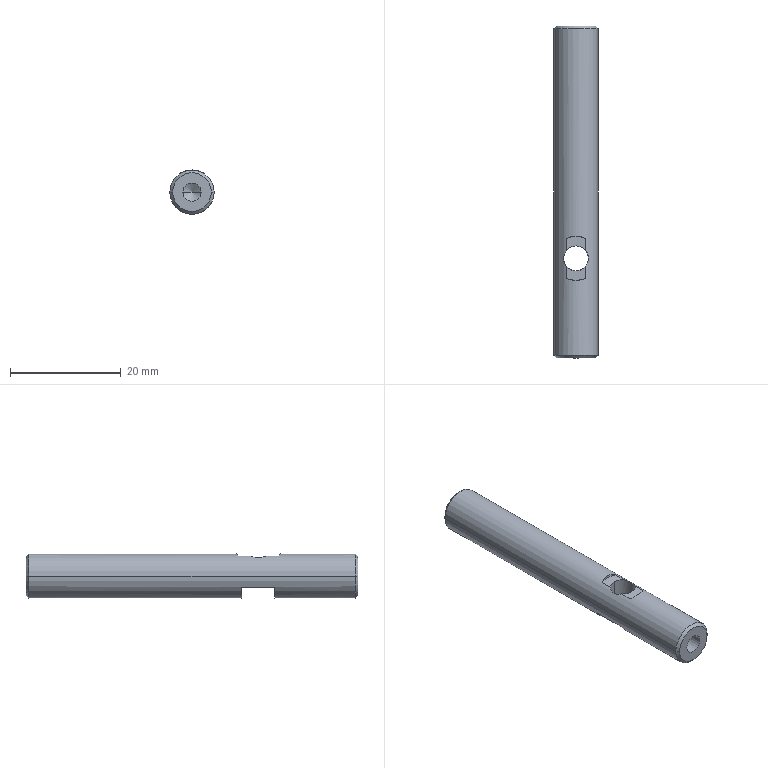Component | SolidWorks | 002MaterialPickingModuleA-1_004SidePlugModule-1_J-017-1 | 1 solid | 26 faces | box 8 x 60 x 8 mm | volume 2727 mm3 | cylinder 11 | cone 8 | plane 7 | commonest cylinder face diameters 8 x5 3.3 x2 4.5 x2 2.5 x2 | material 45
build123d program:
from build123d import *

# Parameters (mm, degrees)
SKETCH1_R             = 4
BOSS_EXTRUDE1_DEPTH   = 48
M3_TAPPED_HOLE1_D     = 2.5
M3_TAPPED_HOLE1_DEPTH = 7.5
M3_TAPPED_HOLE1_TIP   = 0.7511
CHAMFER1_SIZE         = 0.5
SKETCH6_W             = 15
SKETCH6_H             = 6
CUT_EXTRUDE1_DEPTH    = 2
SKETCH9_R             = 4
BOSS_EXTRUDE2_DEPTH   = 12
CHAMFER2_SIZE         = 0.5
M4_TAPPED_HOLE1_D     = 3.3
M4_TAPPED_HOLE1_DEPTH = 10.1
M4_TAPPED_HOLE1_TIP   = 0.9914


with BuildPart() as part:
    # Sketch1 → Boss-Extrude1 (new body)
    with BuildSketch(Plane.XY):
        Circle(SKETCH1_R)
    extrude(amount=BOSS_EXTRUDE1_DEPTH)

    # M3 Tapped Hole1
    with Locations(Plane(origin=(0, 0, 0), x_dir=(-1, 0, 0), z_dir=(0, 0, -1))):
        with Locations((0, 0)):
            Hole(M3_TAPPED_HOLE1_D / 2, depth=M3_TAPPED_HOLE1_DEPTH)
            with Locations((0, 0, -(M3_TAPPED_HOLE1_DEPTH + M3_TAPPED_HOLE1_TIP / 2))):  # 118° drill point
                Cone(0, M3_TAPPED_HOLE1_D / 2, M3_TAPPED_HOLE1_TIP, mode=Mode.SUBTRACT)

    # Chamfer1
    chamfer1_edges = [part.edges().sort_by_distance(p)[0] for p in [
        (-4, 0, 0),
    ]]
    chamfer(chamfer1_edges, length=CHAMFER1_SIZE)

    # Sketch6 → Cut-Extrude1 (cut)
    with BuildSketch(Plane(origin=(0, 4, 0), x_dir=(1, 0, 0), z_dir=(0, 1, 0))):
        with Locations((0, -42)):
            Rectangle(SKETCH6_W, SKETCH6_H)
    extrude(amount=-CUT_EXTRUDE1_DEPTH, mode=Mode.SUBTRACT)

    # Sketch8 → M4 Hex Socket Head Cap Screw CBORE1 (revolve, cut)
    with BuildSketch(Plane(origin=(0, -8, 42), x_dir=(0, 0, -1), z_dir=(1, 0, 0))):
        Polygon((0, 0), (0, 12), (2.25, 12), (2.25, 4.4), (4, 4.4), (4, 0.025), (4.025, 0), align=None)
    revolve(axis=Axis((0, -14.35, 42), (0, 1, 0)), mode=Mode.SUBTRACT)

    # Sketch9 → Boss-Extrude2 (add)
    with BuildSketch(Plane.XY.offset(48)):
        Circle(SKETCH9_R)
    extrude(amount=BOSS_EXTRUDE2_DEPTH)

    # Chamfer2
    chamfer2_edges = [part.edges().sort_by_distance(p)[0] for p in [
        (-4, 0, 60),
    ]]
    chamfer(chamfer2_edges, length=CHAMFER2_SIZE)

    # M4 Tapped Hole1
    with Locations(Plane.XY.offset(60)):
        with Locations((0, 0)):
            Hole(M4_TAPPED_HOLE1_D / 2, depth=M4_TAPPED_HOLE1_DEPTH)
            with Locations((0, 0, -(M4_TAPPED_HOLE1_DEPTH + M4_TAPPED_HOLE1_TIP / 2))):  # 118° drill point
                Cone(0, M4_TAPPED_HOLE1_D / 2, M4_TAPPED_HOLE1_TIP, mode=Mode.SUBTRACT)


solid = part.part

# Placed as in the assembly
solid = solid.moved(Location((195.325, 338.019, 464.731), (90, 0, -180)))
STEP:
#1=CARTESIAN_POINT('',(7.755,11.343,18.296));
#2=VERTEX_POINT('',#1);
#3=CARTESIAN_POINT('',(7.625,11.343,18.296));
#4=VERTEX_POINT('',#3);
#5=CARTESIAN_POINT('',(7.69,11.343,18.296));
#6=DIRECTION('',(0.,-1.,-0.));
#7=DIRECTION('',(-1.,0.,0.));
#8=AXIS2_PLACEMENT_3D('',#5,#6,#7);
#9=CIRCLE('',#8,0.06496);
#10=EDGE_CURVE('',#2,#4,#9,.T.);
#11=ORIENTED_EDGE('',*,*,#10,.F.);
#12=CARTESIAN_POINT('',(7.755,10.946,18.296));
#13=VERTEX_POINT('',#12);
#14=CARTESIAN_POINT('',(7.755,10.946,18.296));
#15=DIRECTION('',(0.,-1.,-0.));
#16=VECTOR('',#15,39.37);
#17=LINE('',#14,#16);
#18=EDGE_CURVE('',#2,#13,#17,.T.);
#19=ORIENTED_EDGE('',*,*,#18,.T.);
#20=CARTESIAN_POINT('',(7.625,10.946,18.296));
#21=VERTEX_POINT('',#20);
#22=CARTESIAN_POINT('',(7.69,10.946,18.296));
#23=DIRECTION('',(0.,-1.,-0.));
#24=DIRECTION('',(-1.,0.,0.));
#25=AXIS2_PLACEMENT_3D('',#22,#23,#24);
#26=CIRCLE('',#25,0.06496);
#27=EDGE_CURVE('',#13,#21,#26,.T.);
#28=ORIENTED_EDGE('',*,*,#27,.T.);
#29=CARTESIAN_POINT('',(7.625,10.946,18.296));
#30=DIRECTION('',(0.,-1.,-0.));
#31=VECTOR('',#30,39.37);
#32=LINE('',#29,#31);
#33=EDGE_CURVE('',#4,#21,#32,.T.);
#34=ORIENTED_EDGE('',*,*,#33,.F.);
#35=EDGE_LOOP('',(#11,#19,#28,#34));
#36=FACE_OUTER_BOUND('',#35,.T.);
#37=CARTESIAN_POINT('',(7.69,10.946,18.296));
#38=DIRECTION('',(0.,-1.,-0.));
#39=DIRECTION('',(-1.,0.,0.));
#40=AXIS2_PLACEMENT_3D('',#37,#38,#39);
#41=CYLINDRICAL_SURFACE('',#40,0.06496);
#42=ADVANCED_FACE('',(#36),#41,.F.);
#43=CARTESIAN_POINT('',(7.69,11.382,18.296));
#44=VERTEX_POINT('',#43);
#45=CARTESIAN_POINT('',(7.625,11.343,18.296));
#46=DIRECTION('',(-0.8572,-0.515,0.));
#47=VECTOR('',#46,39.37);
#48=LINE('',#45,#47);
#49=EDGE_CURVE('',#44,#4,#48,.T.);
#50=ORIENTED_EDGE('',*,*,#49,.F.);
#51=CARTESIAN_POINT('',(7.755,11.343,18.296));
#52=DIRECTION('',(0.8572,-0.515,-0.));
#53=VECTOR('',#52,39.37);
#54=LINE('',#51,#53);
#55=EDGE_CURVE('',#44,#2,#54,.T.);
#56=ORIENTED_EDGE('',*,*,#55,.T.);
#57=ORIENTED_EDGE('',*,*,#10,.T.);
#58=EDGE_LOOP('',(#50,#56,#57));
#59=FACE_OUTER_BOUND('',#58,.T.);
#60=CARTESIAN_POINT('',(7.69,11.343,18.296));
#61=DIRECTION('',(0.,-1.,-0.));
#62=DIRECTION('',(-1.,0.,0.));
#63=AXIS2_PLACEMENT_3D('',#60,#61,#62);
#64=CONICAL_SURFACE('',#63,0.06496,1.03);
#65=ADVANCED_FACE('',(#59),#64,.F.);
#66=CARTESIAN_POINT('',(7.552,10.946,18.296));
#67=VERTEX_POINT('',#66);
#68=CARTESIAN_POINT('',(7.828,10.946,18.296));
#69=VERTEX_POINT('',#68);
#70=CARTESIAN_POINT('',(7.69,10.946,18.296));
#71=DIRECTION('',(0.,-1.,-0.));
#72=DIRECTION('',(-1.,0.,0.));
#73=AXIS2_PLACEMENT_3D('',#70,#71,#72);
#74=CIRCLE('',#73,0.1378);
#75=EDGE_CURVE('',#67,#69,#74,.T.);
#76=ORIENTED_EDGE('',*,*,#75,.F.);
#77=CARTESIAN_POINT('',(7.532,10.965,18.296));
#78=VERTEX_POINT('',#77);
#79=CARTESIAN_POINT('',(7.552,10.946,18.296));
#80=DIRECTION('',(-0.7071,0.7071,0.));
#81=VECTOR('',#80,39.37);
#82=LINE('',#79,#81);
#83=EDGE_CURVE('',#67,#78,#82,.T.);
#84=ORIENTED_EDGE('',*,*,#83,.T.);
#85=CARTESIAN_POINT('',(7.847,10.965,18.296));
#86=VERTEX_POINT('',#85);
#87=CARTESIAN_POINT('',(7.69,10.965,18.296));
#88=DIRECTION('',(-0.,1.,0.));
#89=DIRECTION('',(-1.,0.,0.));
#90=AXIS2_PLACEMENT_3D('',#87,#88,#89);
#91=CIRCLE('',#90,0.1575);
#92=EDGE_CURVE('',#86,#78,#91,.T.);
#93=ORIENTED_EDGE('',*,*,#92,.F.);
#94=CARTESIAN_POINT('',(7.828,10.946,18.296));
#95=DIRECTION('',(0.7071,0.7071,-0.));
#96=VECTOR('',#95,39.37);
#97=LINE('',#94,#96);
#98=EDGE_CURVE('',#69,#86,#97,.T.);
#99=ORIENTED_EDGE('',*,*,#98,.F.);
#100=EDGE_LOOP('',(#76,#84,#93,#99));
#101=FACE_OUTER_BOUND('',#100,.T.);
#102=CARTESIAN_POINT('',(7.69,10.946,18.296));
#103=DIRECTION('',(-0.,1.,0.));
#104=DIRECTION('',(1.,0.,0.));
#105=AXIS2_PLACEMENT_3D('',#102,#103,#104);
#106=CONICAL_SURFACE('',#105,0.1378,0.7854);
#107=ADVANCED_FACE('',(#101),#106,.T.);
#108=CARTESIAN_POINT('',(7.69,11.743,18.218));
#109=VERTEX_POINT('',#108);
#110=CARTESIAN_POINT('',(7.69,11.566,18.218));
#111=VERTEX_POINT('',#110);
#112=CARTESIAN_POINT('',(7.69,11.654,18.218));
#113=DIRECTION('',(-0.,0.,-1.));
#114=DIRECTION('',(0.,-1.,0.));
#115=AXIS2_PLACEMENT_3D('',#112,#113,#114);
#116=CIRCLE('',#115,0.08858);
#117=EDGE_CURVE('',#109,#111,#116,.T.);
#118=ORIENTED_EDGE('',*,*,#117,.T.);
#119=CARTESIAN_POINT('',(7.69,11.566,18.438));
#120=VERTEX_POINT('',#119);
#121=CARTESIAN_POINT('',(7.69,11.566,18.611));
#122=DIRECTION('',(0.,-0.,1.));
#123=VECTOR('',#122,39.37);
#124=LINE('',#121,#123);
#125=EDGE_CURVE('',#111,#120,#124,.T.);
#126=ORIENTED_EDGE('',*,*,#125,.T.);
#127=CARTESIAN_POINT('',(7.759,11.598,18.438));
#128=VERTEX_POINT('',#127);
#129=CARTESIAN_POINT('',(7.69,11.654,18.438));
#130=DIRECTION('',(0.,-0.,1.));
#131=DIRECTION('',(0.,1.,0.));
#132=AXIS2_PLACEMENT_3D('',#129,#130,#131);
#133=CIRCLE('',#132,0.08858);
#134=EDGE_CURVE('',#120,#128,#133,.T.);
#135=ORIENTED_EDGE('',*,*,#134,.T.);
#136=CARTESIAN_POINT('',(7.759,11.71,18.438));
#137=VERTEX_POINT('',#136);
#138=CARTESIAN_POINT('',(7.759,11.71,18.438));
#139=CARTESIAN_POINT('',(7.765,11.703,18.435));
#140=CARTESIAN_POINT('',(7.77,11.694,18.432));
#141=CARTESIAN_POINT('',(7.775,11.68,18.429));
#142=CARTESIAN_POINT('',(7.776,11.675,18.428));
#143=CARTESIAN_POINT('',(7.778,11.665,18.427));
#144=CARTESIAN_POINT('',(7.779,11.66,18.427));
#145=CARTESIAN_POINT('',(7.779,11.649,18.427));
#146=CARTESIAN_POINT('',(7.778,11.644,18.427));
#147=CARTESIAN_POINT('',(7.776,11.634,18.428));
#148=CARTESIAN_POINT('',(7.775,11.629,18.429));
#149=CARTESIAN_POINT('',(7.77,11.615,18.432));
#150=CARTESIAN_POINT('',(7.765,11.606,18.435));
#151=CARTESIAN_POINT('',(7.759,11.598,18.438));
#152=B_SPLINE_CURVE_WITH_KNOTS('',3,(#138,#139,#140,#141,#142,#143,#144,#145,#146,#147,#148,#149,#150,#151),.UNSPECIFIED.,.F.,.F.,(4,2,2,2,2,2,4),(0.,0.0007826,0.001174,0.001565,0.001957,0.002348,0.00313),.UNSPECIFIED.);
#153=EDGE_CURVE('',#137,#128,#152,.T.);
#154=ORIENTED_EDGE('',*,*,#153,.F.);
#155=CARTESIAN_POINT('',(7.69,11.743,18.438));
#156=VERTEX_POINT('',#155);
#157=CARTESIAN_POINT('',(7.69,11.654,18.438));
#158=DIRECTION('',(0.,-0.,1.));
#159=DIRECTION('',(0.,1.,0.));
#160=AXIS2_PLACEMENT_3D('',#157,#158,#159);
#161=CIRCLE('',#160,0.08858);
#162=EDGE_CURVE('',#137,#156,#161,.T.);
#163=ORIENTED_EDGE('',*,*,#162,.T.);
#164=CARTESIAN_POINT('',(7.69,11.743,18.611));
#165=DIRECTION('',(0.,-0.,1.));
#166=VECTOR('',#165,39.37);
#167=LINE('',#164,#166);
#168=EDGE_CURVE('',#109,#156,#167,.T.);
#169=ORIENTED_EDGE('',*,*,#168,.F.);
#170=EDGE_LOOP('',(#118,#126,#135,#154,#163,#169));
#171=FACE_OUTER_BOUND('',#170,.T.);
#172=CARTESIAN_POINT('',(7.69,11.654,18.611));
#173=DIRECTION('',(0.,-0.,1.));
#174=DIRECTION('',(0.,1.,0.));
#175=AXIS2_PLACEMENT_3D('',#172,#173,#174);
#176=CYLINDRICAL_SURFACE('',#175,0.08858);
#177=ADVANCED_FACE('',(#171),#176,.F.);
#178=CARTESIAN_POINT('',(7.69,11.812,18.438));
#179=VERTEX_POINT('',#178);
#180=CARTESIAN_POINT('',(7.621,11.796,18.438));
#181=VERTEX_POINT('',#180);
#182=CARTESIAN_POINT('',(7.69,11.654,18.438));
#183=DIRECTION('',(0.,-0.,1.));
#184=DIRECTION('',(0.,1.,0.));
#185=AXIS2_PLACEMENT_3D('',#182,#183,#184);
#186=CIRCLE('',#185,0.1575);
#187=EDGE_CURVE('',#179,#181,#186,.T.);
#188=ORIENTED_EDGE('',*,*,#187,.F.);
#189=CARTESIAN_POINT('',(7.69,11.812,18.454));
#190=VERTEX_POINT('',#189);
#191=CARTESIAN_POINT('',(7.69,11.812,18.611));
#192=DIRECTION('',(0.,-0.,1.));
#193=VECTOR('',#192,39.37);
#194=LINE('',#191,#193);
#195=EDGE_CURVE('',#179,#190,#194,.T.);
#196=ORIENTED_EDGE('',*,*,#195,.T.);
#197=CARTESIAN_POINT('',(7.621,11.796,18.438));
#198=CARTESIAN_POINT('',(7.643,11.806,18.449));
#199=CARTESIAN_POINT('',(7.666,11.812,18.454));
#200=CARTESIAN_POINT('',(7.69,11.812,18.454));
#201=(BOUNDED_CURVE()B_SPLINE_CURVE(3,(#197,#198,#199,#200),.UNSPECIFIED.,.F.,.T.)B_SPLINE_CURVE_WITH_KNOTS((4,4),(5.832,6.283),.UNSPECIFIED.)CURVE()GEOMETRIC_REPRESENTATION_ITEM()RATIONAL_B_SPLINE_CURVE((1.,0.9831,0.9831,1.))REPRESENTATION_ITEM(''));
#202=EDGE_CURVE('',#181,#190,#201,.T.);
#203=ORIENTED_EDGE('',*,*,#202,.F.);
#204=EDGE_LOOP('',(#188,#196,#203));
#205=FACE_OUTER_BOUND('',#204,.T.);
#206=CARTESIAN_POINT('',(7.69,11.654,18.611));
#207=DIRECTION('',(0.,-0.,1.));
#208=DIRECTION('',(0.,1.,0.));
#209=AXIS2_PLACEMENT_3D('',#206,#207,#208);
#210=CYLINDRICAL_SURFACE('',#209,0.1575);
#211=ADVANCED_FACE('',(#205),#210,.F.);
#212=CARTESIAN_POINT('',(7.828,13.308,18.296));
#213=VERTEX_POINT('',#212);
#214=CARTESIAN_POINT('',(7.552,13.308,18.296));
#215=VERTEX_POINT('',#214);
#216=CARTESIAN_POINT('',(7.69,13.308,18.296));
#217=DIRECTION('',(-0.,1.,0.));
#218=DIRECTION('',(-1.,0.,0.));
#219=AXIS2_PLACEMENT_3D('',#216,#217,#218);
#220=CIRCLE('',#219,0.1378);
#221=EDGE_CURVE('',#213,#215,#220,.T.);
#222=ORIENTED_EDGE('',*,*,#221,.F.);
#223=CARTESIAN_POINT('',(7.847,13.288,18.296));
#224=VERTEX_POINT('',#223);
#225=CARTESIAN_POINT('',(7.847,13.288,18.296));
#226=DIRECTION('',(0.7071,-0.7071,-0.));
#227=VECTOR('',#226,39.37);
#228=LINE('',#225,#227);
#229=EDGE_CURVE('',#213,#224,#228,.T.);
#230=ORIENTED_EDGE('',*,*,#229,.T.);
#231=CARTESIAN_POINT('',(7.532,13.288,18.296));
#232=VERTEX_POINT('',#231);
#233=CARTESIAN_POINT('',(7.69,13.288,18.296));
#234=DIRECTION('',(0.,-1.,-0.));
#235=DIRECTION('',(-1.,0.,0.));
#236=AXIS2_PLACEMENT_3D('',#233,#234,#235);
#237=CIRCLE('',#236,0.1575);
#238=EDGE_CURVE('',#232,#224,#237,.T.);
#239=ORIENTED_EDGE('',*,*,#238,.F.);
#240=CARTESIAN_POINT('',(7.532,13.288,18.296));
#241=DIRECTION('',(-0.7071,-0.7071,0.));
#242=VECTOR('',#241,39.37);
#243=LINE('',#240,#242);
#244=EDGE_CURVE('',#215,#232,#243,.T.);
#245=ORIENTED_EDGE('',*,*,#244,.F.);
#246=EDGE_LOOP('',(#222,#230,#239,#245));
#247=FACE_OUTER_BOUND('',#246,.T.);
#248=CARTESIAN_POINT('',(7.69,13.288,18.296));
#249=DIRECTION('',(0.,-1.,-0.));
#250=DIRECTION('',(-1.,0.,0.));
#251=AXIS2_PLACEMENT_3D('',#248,#249,#250);
#252=CONICAL_SURFACE('',#251,0.1575,0.7854);
#253=ADVANCED_FACE('',(#247),#252,.T.);
#254=CARTESIAN_POINT('',(7.641,13.013,18.296));
#255=VERTEX_POINT('',#254);
#256=CARTESIAN_POINT('',(7.739,13.013,18.296));
#257=VERTEX_POINT('',#256);
#258=CARTESIAN_POINT('',(7.69,13.013,18.296));
#259=DIRECTION('',(-0.,1.,0.));
#260=DIRECTION('',(1.,0.,0.));
#261=AXIS2_PLACEMENT_3D('',#258,#259,#260);
#262=CIRCLE('',#261,0.04921);
#263=EDGE_CURVE('',#255,#257,#262,.T.);
#264=ORIENTED_EDGE('',*,*,#263,.F.);
#265=CARTESIAN_POINT('',(7.641,13.308,18.296));
#266=VERTEX_POINT('',#265);
#267=CARTESIAN_POINT('',(7.641,13.308,18.296));
#268=DIRECTION('',(-0.,1.,0.));
#269=VECTOR('',#268,39.37);
#270=LINE('',#267,#269);
#271=EDGE_CURVE('',#255,#266,#270,.T.);
#272=ORIENTED_EDGE('',*,*,#271,.T.);
#273=CARTESIAN_POINT('',(7.739,13.308,18.296));
#274=VERTEX_POINT('',#273);
#275=CARTESIAN_POINT('',(7.69,13.308,18.296));
#276=DIRECTION('',(-0.,1.,0.));
#277=DIRECTION('',(1.,0.,0.));
#278=AXIS2_PLACEMENT_3D('',#275,#276,#277);
#279=CIRCLE('',#278,0.04921);
#280=EDGE_CURVE('',#266,#274,#279,.T.);
#281=ORIENTED_EDGE('',*,*,#280,.T.);
#282=CARTESIAN_POINT('',(7.739,13.308,18.296));
#283=DIRECTION('',(-0.,1.,0.));
#284=VECTOR('',#283,39.37);
#285=LINE('',#282,#284);
#286=EDGE_CURVE('',#257,#274,#285,.T.);
#287=ORIENTED_EDGE('',*,*,#286,.F.);
#288=EDGE_LOOP('',(#264,#272,#281,#287));
#289=FACE_OUTER_BOUND('',#288,.T.);
#290=CARTESIAN_POINT('',(7.69,13.308,18.296));
#291=DIRECTION('',(-0.,1.,0.));
#292=DIRECTION('',(1.,0.,0.));
#293=AXIS2_PLACEMENT_3D('',#290,#291,#292);
#294=CYLINDRICAL_SURFACE('',#293,0.04921);
#295=ADVANCED_FACE('',(#289),#294,.F.);
#296=CARTESIAN_POINT('',(7.69,12.983,18.296));
#297=VERTEX_POINT('',#296);
#298=CARTESIAN_POINT('',(7.739,13.013,18.296));
#299=DIRECTION('',(0.8572,0.515,-0.));
#300=VECTOR('',#299,39.37);
#301=LINE('',#298,#300);
#302=EDGE_CURVE('',#297,#257,#301,.T.);
#303=ORIENTED_EDGE('',*,*,#302,.F.);
#304=CARTESIAN_POINT('',(7.641,13.013,18.296));
#305=DIRECTION('',(-0.8572,0.515,0.));
#306=VECTOR('',#305,39.37);
#307=LINE('',#304,#306);
#308=EDGE_CURVE('',#297,#255,#307,.T.);
#309=ORIENTED_EDGE('',*,*,#308,.T.);
#310=ORIENTED_EDGE('',*,*,#263,.T.);
#311=EDGE_LOOP('',(#303,#309,#310));
#312=FACE_OUTER_BOUND('',#311,.T.);
#313=CARTESIAN_POINT('',(7.69,13.013,18.296));
#314=DIRECTION('',(-0.,1.,0.));
#315=DIRECTION('',(1.,0.,0.));
#316=AXIS2_PLACEMENT_3D('',#313,#314,#315);
#317=CONICAL_SURFACE('',#316,0.04921,1.03);
#318=ADVANCED_FACE('',(#312),#317,.F.);
#319=CARTESIAN_POINT('',(7.826,11.772,18.218));
#320=VERTEX_POINT('',#319);
#321=CARTESIAN_POINT('',(7.826,11.536,18.218));
#322=VERTEX_POINT('',#321);
#323=CARTESIAN_POINT('',(7.826,11.418,18.218));
#324=DIRECTION('',(0.,-1.,-0.));
#325=VECTOR('',#324,39.37);
#326=LINE('',#323,#325);
#327=EDGE_CURVE('',#320,#322,#326,.T.);
#328=ORIENTED_EDGE('',*,*,#327,.F.);
#329=CARTESIAN_POINT('',(7.554,11.772,18.218));
#330=VERTEX_POINT('',#329);
#331=CARTESIAN_POINT('',(7.69,11.772,18.296));
#332=DIRECTION('',(-0.,1.,0.));
#333=DIRECTION('',(1.,0.,0.));
#334=AXIS2_PLACEMENT_3D('',#331,#332,#333);
#335=CIRCLE('',#334,0.1575);
#336=EDGE_CURVE('',#320,#330,#335,.T.);
#337=ORIENTED_EDGE('',*,*,#336,.T.);
#338=CARTESIAN_POINT('',(7.554,11.536,18.218));
#339=VERTEX_POINT('',#338);
#340=CARTESIAN_POINT('',(7.554,11.418,18.218));
#341=DIRECTION('',(-0.,1.,0.));
#342=VECTOR('',#341,39.37);
#343=LINE('',#340,#342);
#344=EDGE_CURVE('',#339,#330,#343,.T.);
#345=ORIENTED_EDGE('',*,*,#344,.F.);
#346=CARTESIAN_POINT('',(7.69,11.536,18.296));
#347=DIRECTION('',(0.,-1.,-0.));
#348=DIRECTION('',(-1.,0.,0.));
#349=AXIS2_PLACEMENT_3D('',#346,#347,#348);
#350=CIRCLE('',#349,0.1575);
#351=EDGE_CURVE('',#339,#322,#350,.T.);
#352=ORIENTED_EDGE('',*,*,#351,.T.);
#353=EDGE_LOOP('',(#328,#337,#345,#352));
#354=FACE_BOUND('',#353,.T.);
#355=ORIENTED_EDGE('',*,*,#92,.T.);
#356=CARTESIAN_POINT('',(7.532,11.418,18.296));
#357=DIRECTION('',(-0.,1.,0.));
#358=VECTOR('',#357,39.37);
#359=LINE('',#356,#358);
#360=EDGE_CURVE('',#78,#232,#359,.T.);
#361=ORIENTED_EDGE('',*,*,#360,.T.);
#362=ORIENTED_EDGE('',*,*,#238,.T.);
#363=CARTESIAN_POINT('',(7.847,11.418,18.296));
#364=DIRECTION('',(-0.,1.,0.));
#365=VECTOR('',#364,39.37);
#366=LINE('',#363,#365);
#367=EDGE_CURVE('',#86,#224,#366,.T.);
#368=ORIENTED_EDGE('',*,*,#367,.F.);
#369=EDGE_LOOP('',(#355,#361,#362,#368));
#370=FACE_OUTER_BOUND('',#369,.T.);
#371=CARTESIAN_POINT('',(7.69,11.418,18.296));
#372=DIRECTION('',(-0.,1.,0.));
#373=DIRECTION('',(1.,0.,0.));
#374=AXIS2_PLACEMENT_3D('',#371,#372,#373);
#375=CYLINDRICAL_SURFACE('',#374,0.1575);
#376=ADVANCED_FACE('',(#354,#370),#375,.T.);
#377=ORIENTED_EDGE('',*,*,#360,.F.);
#378=CARTESIAN_POINT('',(7.69,10.965,18.296));
#379=DIRECTION('',(-0.,1.,0.));
#380=DIRECTION('',(-1.,0.,0.));
#381=AXIS2_PLACEMENT_3D('',#378,#379,#380);
#382=CIRCLE('',#381,0.1575);
#383=EDGE_CURVE('',#78,#86,#382,.T.);
#384=ORIENTED_EDGE('',*,*,#383,.T.);
#385=ORIENTED_EDGE('',*,*,#367,.T.);
#386=CARTESIAN_POINT('',(7.69,13.288,18.296));
#387=DIRECTION('',(0.,-1.,-0.));
#388=DIRECTION('',(-1.,0.,0.));
#389=AXIS2_PLACEMENT_3D('',#386,#387,#388);
#390=CIRCLE('',#389,0.1575);
#391=EDGE_CURVE('',#224,#232,#390,.T.);
#392=ORIENTED_EDGE('',*,*,#391,.T.);
#393=EDGE_LOOP('',(#377,#384,#385,#392));
#394=FACE_OUTER_BOUND('',#393,.T.);
#395=CARTESIAN_POINT('',(7.621,11.513,18.438));
#396=VERTEX_POINT('',#395);
#397=CARTESIAN_POINT('',(7.621,11.598,18.438));
#398=VERTEX_POINT('',#397);
#399=CARTESIAN_POINT('',(7.621,11.418,18.438));
#400=DIRECTION('',(-0.,1.,0.));
#401=VECTOR('',#400,39.37);
#402=LINE('',#399,#401);
#403=EDGE_CURVE('',#396,#398,#402,.T.);
#404=ORIENTED_EDGE('',*,*,#403,.T.);
#405=CARTESIAN_POINT('',(7.621,11.71,18.438));
#406=VERTEX_POINT('',#405);
#407=CARTESIAN_POINT('',(7.621,11.598,18.438));
#408=CARTESIAN_POINT('',(7.615,11.606,18.435));
#409=CARTESIAN_POINT('',(7.61,11.615,18.432));
#410=CARTESIAN_POINT('',(7.605,11.629,18.429));
#411=CARTESIAN_POINT('',(7.604,11.634,18.428));
#412=CARTESIAN_POINT('',(7.602,11.644,18.427));
#413=CARTESIAN_POINT('',(7.601,11.649,18.427));
#414=CARTESIAN_POINT('',(7.601,11.659,18.427));
#415=CARTESIAN_POINT('',(7.602,11.664,18.427));
#416=CARTESIAN_POINT('',(7.604,11.675,18.428));
#417=CARTESIAN_POINT('',(7.605,11.68,18.429));
#418=CARTESIAN_POINT('',(7.61,11.694,18.432));
#419=CARTESIAN_POINT('',(7.615,11.703,18.435));
#420=CARTESIAN_POINT('',(7.621,11.71,18.438));
#421=B_SPLINE_CURVE_WITH_KNOTS('',3,(#407,#408,#409,#410,#411,#412,#413,#414,#415,#416,#417,#418,#419,#420),.UNSPECIFIED.,.F.,.F.,(4,2,2,2,2,2,4),(0.,0.0007826,0.001174,0.001565,0.001957,0.002348,0.00313),.UNSPECIFIED.);
#422=EDGE_CURVE('',#398,#406,#421,.T.);
#423=ORIENTED_EDGE('',*,*,#422,.T.);
#424=CARTESIAN_POINT('',(7.621,11.418,18.438));
#425=DIRECTION('',(-0.,1.,0.));
#426=VECTOR('',#425,39.37);
#427=LINE('',#424,#426);
#428=EDGE_CURVE('',#406,#181,#427,.T.);
#429=ORIENTED_EDGE('',*,*,#428,.T.);
#430=ORIENTED_EDGE('',*,*,#202,.T.);
#431=CARTESIAN_POINT('',(7.759,11.796,18.438));
#432=VERTEX_POINT('',#431);
#433=CARTESIAN_POINT('',(7.69,11.812,18.454));
#434=CARTESIAN_POINT('',(7.714,11.812,18.454));
#435=CARTESIAN_POINT('',(7.737,11.806,18.449));
#436=CARTESIAN_POINT('',(7.759,11.796,18.438));
#437=(BOUNDED_CURVE()B_SPLINE_CURVE(3,(#433,#434,#435,#436),.UNSPECIFIED.,.F.,.F.)B_SPLINE_CURVE_WITH_KNOTS((4,4),(0.,0.451),.UNSPECIFIED.)CURVE()GEOMETRIC_REPRESENTATION_ITEM()RATIONAL_B_SPLINE_CURVE((1.,0.9831,0.9831,1.))REPRESENTATION_ITEM(''));
#438=EDGE_CURVE('',#190,#432,#437,.T.);
#439=ORIENTED_EDGE('',*,*,#438,.T.);
#440=CARTESIAN_POINT('',(7.759,11.418,18.438));
#441=DIRECTION('',(0.,-1.,-0.));
#442=VECTOR('',#441,39.37);
#443=LINE('',#440,#442);
#444=EDGE_CURVE('',#432,#137,#443,.T.);
#445=ORIENTED_EDGE('',*,*,#444,.T.);
#446=ORIENTED_EDGE('',*,*,#153,.T.);
#447=CARTESIAN_POINT('',(7.759,11.513,18.438));
#448=VERTEX_POINT('',#447);
#449=CARTESIAN_POINT('',(7.759,11.418,18.438));
#450=DIRECTION('',(0.,-1.,-0.));
#451=VECTOR('',#450,39.37);
#452=LINE('',#449,#451);
#453=EDGE_CURVE('',#128,#448,#452,.T.);
#454=ORIENTED_EDGE('',*,*,#453,.T.);
#455=CARTESIAN_POINT('',(7.759,11.513,18.438));
#456=CARTESIAN_POINT('',(7.714,11.491,18.46));
#457=CARTESIAN_POINT('',(7.665,11.491,18.46));
#458=CARTESIAN_POINT('',(7.621,11.513,18.438));
#459=(BOUNDED_CURVE()B_SPLINE_CURVE(3,(#455,#456,#457,#458),.UNSPECIFIED.,.F.,.F.)B_SPLINE_CURVE_WITH_KNOTS((4,4),(2.691,3.593),.UNSPECIFIED.)CURVE()GEOMETRIC_REPRESENTATION_ITEM()RATIONAL_B_SPLINE_CURVE((1.,0.9333,0.9333,1.))REPRESENTATION_ITEM(''));
#460=EDGE_CURVE('',#448,#396,#459,.T.);
#461=ORIENTED_EDGE('',*,*,#460,.T.);
#462=EDGE_LOOP('',(#404,#423,#429,#430,#439,#445,#446,#454,#461));
#463=FACE_BOUND('',#462,.T.);
#464=CARTESIAN_POINT('',(7.69,11.418,18.296));
#465=DIRECTION('',(-0.,1.,0.));
#466=DIRECTION('',(1.,0.,0.));
#467=AXIS2_PLACEMENT_3D('',#464,#465,#466);
#468=CYLINDRICAL_SURFACE('',#467,0.1575);
#469=ADVANCED_FACE('',(#394,#463),#468,.T.);
#470=CARTESIAN_POINT('',(7.69,13.308,18.296));
#471=DIRECTION('',(-0.,1.,0.));
#472=DIRECTION('',(-1.,0.,0.));
#473=AXIS2_PLACEMENT_3D('',#470,#471,#472);
#474=CIRCLE('',#473,0.1378);
#475=EDGE_CURVE('',#215,#213,#474,.T.);
#476=ORIENTED_EDGE('',*,*,#475,.T.);
#477=ORIENTED_EDGE('',*,*,#221,.T.);
#478=EDGE_LOOP('',(#476,#477));
#479=FACE_OUTER_BOUND('',#478,.T.);
#480=CARTESIAN_POINT('',(7.69,13.308,18.296));
#481=DIRECTION('',(-0.,1.,0.));
#482=DIRECTION('',(1.,0.,0.));
#483=AXIS2_PLACEMENT_3D('',#480,#481,#482);
#484=CIRCLE('',#483,0.04921);
#485=EDGE_CURVE('',#274,#266,#484,.T.);
#486=ORIENTED_EDGE('',*,*,#485,.F.);
#487=ORIENTED_EDGE('',*,*,#280,.F.);
#488=EDGE_LOOP('',(#486,#487));
#489=FACE_BOUND('',#488,.T.);
#490=CARTESIAN_POINT('',(7.69,13.308,18.296));
#491=DIRECTION('',(0.,-1.,-0.));
#492=DIRECTION('',(-1.,-0.,0.));
#493=AXIS2_PLACEMENT_3D('',#490,#491,#492);
#494=PLANE('',#493);
#495=ADVANCED_FACE('',(#479,#489),#494,.F.);
#496=ORIENTED_EDGE('',*,*,#308,.F.);
#497=ORIENTED_EDGE('',*,*,#302,.T.);
#498=CARTESIAN_POINT('',(7.69,13.013,18.296));
#499=DIRECTION('',(-0.,1.,0.));
#500=DIRECTION('',(1.,0.,0.));
#501=AXIS2_PLACEMENT_3D('',#498,#499,#500);
#502=CIRCLE('',#501,0.04921);
#503=EDGE_CURVE('',#257,#255,#502,.T.);
#504=ORIENTED_EDGE('',*,*,#503,.T.);
#505=EDGE_LOOP('',(#496,#497,#504));
#506=FACE_OUTER_BOUND('',#505,.T.);
#507=CARTESIAN_POINT('',(7.69,13.013,18.296));
#508=DIRECTION('',(-0.,1.,0.));
#509=DIRECTION('',(1.,0.,0.));
#510=AXIS2_PLACEMENT_3D('',#507,#508,#509);
#511=CONICAL_SURFACE('',#510,0.04921,1.03);
#512=ADVANCED_FACE('',(#506),#511,.F.);
#513=ORIENTED_EDGE('',*,*,#271,.F.);
#514=ORIENTED_EDGE('',*,*,#503,.F.);
#515=ORIENTED_EDGE('',*,*,#286,.T.);
#516=ORIENTED_EDGE('',*,*,#485,.T.);
#517=EDGE_LOOP('',(#513,#514,#515,#516));
#518=FACE_OUTER_BOUND('',#517,.T.);
#519=CARTESIAN_POINT('',(7.69,13.308,18.296));
#520=DIRECTION('',(-0.,1.,0.));
#521=DIRECTION('',(1.,0.,0.));
#522=AXIS2_PLACEMENT_3D('',#519,#520,#521);
#523=CYLINDRICAL_SURFACE('',#522,0.04921);
#524=ADVANCED_FACE('',(#518),#523,.F.);
#525=ORIENTED_EDGE('',*,*,#229,.F.);
#526=ORIENTED_EDGE('',*,*,#475,.F.);
#527=ORIENTED_EDGE('',*,*,#244,.T.);
#528=ORIENTED_EDGE('',*,*,#391,.F.);
#529=EDGE_LOOP('',(#525,#526,#527,#528));
#530=FACE_OUTER_BOUND('',#529,.T.);
#531=CARTESIAN_POINT('',(7.69,13.288,18.296));
#532=DIRECTION('',(0.,-1.,-0.));
#533=DIRECTION('',(-1.,0.,0.));
#534=AXIS2_PLACEMENT_3D('',#531,#532,#533);
#535=CONICAL_SURFACE('',#534,0.1575,0.7854);
#536=ADVANCED_FACE('',(#530),#535,.T.);
#537=CARTESIAN_POINT('',(7.395,11.772,18.218));
#538=DIRECTION('',(1.,0.,-0.));
#539=VECTOR('',#538,39.37);
#540=LINE('',#537,#539);
#541=EDGE_CURVE('',#330,#320,#540,.T.);
#542=ORIENTED_EDGE('',*,*,#541,.F.);
#543=ORIENTED_EDGE('',*,*,#336,.F.);
#544=EDGE_LOOP('',(#542,#543));
#545=FACE_OUTER_BOUND('',#544,.T.);
#546=CARTESIAN_POINT('',(7.395,11.772,18.218));
#547=DIRECTION('',(-0.,1.,0.));
#548=DIRECTION('',(1.,0.,-0.));
#549=AXIS2_PLACEMENT_3D('',#546,#547,#548);
#550=PLANE('',#549);
#551=ADVANCED_FACE('',(#545),#550,.F.);
#552=CARTESIAN_POINT('',(7.395,11.536,18.218));
#553=DIRECTION('',(-1.,-0.,0.));
#554=VECTOR('',#553,39.37);
#555=LINE('',#552,#554);
#556=EDGE_CURVE('',#322,#339,#555,.T.);
#557=ORIENTED_EDGE('',*,*,#556,.F.);
#558=ORIENTED_EDGE('',*,*,#351,.F.);
#559=EDGE_LOOP('',(#557,#558));
#560=FACE_OUTER_BOUND('',#559,.T.);
#561=CARTESIAN_POINT('',(7.395,11.536,18.218));
#562=DIRECTION('',(0.,-1.,-0.));
#563=DIRECTION('',(-1.,-0.,0.));
#564=AXIS2_PLACEMENT_3D('',#561,#562,#563);
#565=PLANE('',#564);
#566=ADVANCED_FACE('',(#560),#565,.F.);
#567=ORIENTED_EDGE('',*,*,#117,.F.);
#568=CARTESIAN_POINT('',(7.69,11.654,18.218));
#569=DIRECTION('',(-0.,0.,-1.));
#570=DIRECTION('',(0.,-1.,0.));
#571=AXIS2_PLACEMENT_3D('',#568,#569,#570);
#572=CIRCLE('',#571,0.08858);
#573=EDGE_CURVE('',#111,#109,#572,.T.);
#574=ORIENTED_EDGE('',*,*,#573,.F.);
#575=EDGE_LOOP('',(#567,#574));
#576=FACE_BOUND('',#575,.T.);
#577=ORIENTED_EDGE('',*,*,#344,.T.);
#578=ORIENTED_EDGE('',*,*,#541,.T.);
#579=ORIENTED_EDGE('',*,*,#327,.T.);
#580=ORIENTED_EDGE('',*,*,#556,.T.);
#581=EDGE_LOOP('',(#577,#578,#579,#580));
#582=FACE_OUTER_BOUND('',#581,.T.);
#583=CARTESIAN_POINT('',(7.69,13.308,18.218));
#584=DIRECTION('',(-0.,0.,-1.));
#585=DIRECTION('',(0.,-1.,-0.));
#586=AXIS2_PLACEMENT_3D('',#583,#584,#585);
#587=PLANE('',#586);
#588=ADVANCED_FACE('',(#576,#582),#587,.T.);
#589=CARTESIAN_POINT('',(7.69,11.654,18.438));
#590=DIRECTION('',(0.,-0.,1.));
#591=DIRECTION('',(0.,1.,0.));
#592=AXIS2_PLACEMENT_3D('',#589,#590,#591);
#593=CIRCLE('',#592,0.1575);
#594=EDGE_CURVE('',#396,#448,#593,.T.);
#595=ORIENTED_EDGE('',*,*,#594,.T.);
#596=ORIENTED_EDGE('',*,*,#453,.F.);
#597=ORIENTED_EDGE('',*,*,#134,.F.);
#598=CARTESIAN_POINT('',(7.69,11.654,18.438));
#599=DIRECTION('',(0.,-0.,1.));
#600=DIRECTION('',(0.,1.,0.));
#601=AXIS2_PLACEMENT_3D('',#598,#599,#600);
#602=CIRCLE('',#601,0.08858);
#603=EDGE_CURVE('',#398,#120,#602,.T.);
#604=ORIENTED_EDGE('',*,*,#603,.F.);
#605=ORIENTED_EDGE('',*,*,#403,.F.);
#606=EDGE_LOOP('',(#595,#596,#597,#604,#605));
#607=FACE_OUTER_BOUND('',#606,.T.);
#608=CARTESIAN_POINT('',(7.532,11.654,18.438));
#609=DIRECTION('',(-0.,0.,-1.));
#610=DIRECTION('',(0.,-1.,-0.));
#611=AXIS2_PLACEMENT_3D('',#608,#609,#610);
#612=PLANE('',#611);
#613=ADVANCED_FACE('',(#607),#612,.F.);
#614=ORIENTED_EDGE('',*,*,#162,.F.);
#615=ORIENTED_EDGE('',*,*,#444,.F.);
#616=CARTESIAN_POINT('',(7.69,11.654,18.438));
#617=DIRECTION('',(0.,-0.,1.));
#618=DIRECTION('',(0.,1.,0.));
#619=AXIS2_PLACEMENT_3D('',#616,#617,#618);
#620=CIRCLE('',#619,0.1575);
#621=EDGE_CURVE('',#432,#179,#620,.T.);
#622=ORIENTED_EDGE('',*,*,#621,.T.);
#623=ORIENTED_EDGE('',*,*,#187,.T.);
#624=ORIENTED_EDGE('',*,*,#428,.F.);
#625=CARTESIAN_POINT('',(7.69,11.654,18.438));
#626=DIRECTION('',(0.,-0.,1.));
#627=DIRECTION('',(0.,1.,0.));
#628=AXIS2_PLACEMENT_3D('',#625,#626,#627);
#629=CIRCLE('',#628,0.08858);
#630=EDGE_CURVE('',#156,#406,#629,.T.);
#631=ORIENTED_EDGE('',*,*,#630,.F.);
#632=EDGE_LOOP('',(#614,#615,#622,#623,#624,#631));
#633=FACE_OUTER_BOUND('',#632,.T.);
#634=CARTESIAN_POINT('',(7.532,11.654,18.438));
#635=DIRECTION('',(-0.,0.,-1.));
#636=DIRECTION('',(0.,-1.,-0.));
#637=AXIS2_PLACEMENT_3D('',#634,#635,#636);
#638=PLANE('',#637);
#639=ADVANCED_FACE('',(#633),#638,.F.);
#640=ORIENTED_EDGE('',*,*,#594,.F.);
#641=ORIENTED_EDGE('',*,*,#460,.F.);
#642=EDGE_LOOP('',(#640,#641));
#643=FACE_OUTER_BOUND('',#642,.T.);
#644=CARTESIAN_POINT('',(7.69,11.654,18.611));
#645=DIRECTION('',(0.,-0.,1.));
#646=DIRECTION('',(0.,1.,0.));
#647=AXIS2_PLACEMENT_3D('',#644,#645,#646);
#648=CYLINDRICAL_SURFACE('',#647,0.1575);
#649=ADVANCED_FACE('',(#643),#648,.F.);
#650=ORIENTED_EDGE('',*,*,#195,.F.);
#651=ORIENTED_EDGE('',*,*,#621,.F.);
#652=ORIENTED_EDGE('',*,*,#438,.F.);
#653=EDGE_LOOP('',(#650,#651,#652));
#654=FACE_OUTER_BOUND('',#653,.T.);
#655=CARTESIAN_POINT('',(7.69,11.654,18.611));
#656=DIRECTION('',(0.,-0.,1.));
#657=DIRECTION('',(0.,1.,0.));
#658=AXIS2_PLACEMENT_3D('',#655,#656,#657);
#659=CYLINDRICAL_SURFACE('',#658,0.1575);
#660=ADVANCED_FACE('',(#654),#659,.F.);
#661=ORIENTED_EDGE('',*,*,#125,.F.);
#662=ORIENTED_EDGE('',*,*,#573,.T.);
#663=ORIENTED_EDGE('',*,*,#168,.T.);
#664=ORIENTED_EDGE('',*,*,#630,.T.);
#665=ORIENTED_EDGE('',*,*,#422,.F.);
#666=ORIENTED_EDGE('',*,*,#603,.T.);
#667=EDGE_LOOP('',(#661,#662,#663,#664,#665,#666));
#668=FACE_OUTER_BOUND('',#667,.T.);
#669=CARTESIAN_POINT('',(7.69,11.654,18.611));
#670=DIRECTION('',(0.,-0.,1.));
#671=DIRECTION('',(0.,1.,0.));
#672=AXIS2_PLACEMENT_3D('',#669,#670,#671);
#673=CYLINDRICAL_SURFACE('',#672,0.08858);
#674=ADVANCED_FACE('',(#668),#673,.F.);
#675=CARTESIAN_POINT('',(7.69,10.946,18.296));
#676=DIRECTION('',(0.,-1.,-0.));
#677=DIRECTION('',(-1.,0.,0.));
#678=AXIS2_PLACEMENT_3D('',#675,#676,#677);
#679=CIRCLE('',#678,0.06496);
#680=EDGE_CURVE('',#21,#13,#679,.T.);
#681=ORIENTED_EDGE('',*,*,#680,.F.);
#682=ORIENTED_EDGE('',*,*,#27,.F.);
#683=EDGE_LOOP('',(#681,#682));
#684=FACE_BOUND('',#683,.T.);
#685=CARTESIAN_POINT('',(7.69,10.946,18.296));
#686=DIRECTION('',(0.,-1.,-0.));
#687=DIRECTION('',(-1.,0.,0.));
#688=AXIS2_PLACEMENT_3D('',#685,#686,#687);
#689=CIRCLE('',#688,0.1378);
#690=EDGE_CURVE('',#69,#67,#689,.T.);
#691=ORIENTED_EDGE('',*,*,#690,.T.);
#692=ORIENTED_EDGE('',*,*,#75,.T.);
#693=EDGE_LOOP('',(#691,#692));
#694=FACE_OUTER_BOUND('',#693,.T.);
#695=CARTESIAN_POINT('',(7.69,10.946,18.296));
#696=DIRECTION('',(0.,-1.,-0.));
#697=DIRECTION('',(-1.,-0.,0.));
#698=AXIS2_PLACEMENT_3D('',#695,#696,#697);
#699=PLANE('',#698);
#700=ADVANCED_FACE('',(#684,#694),#699,.T.);
#701=ORIENTED_EDGE('',*,*,#83,.F.);
#702=ORIENTED_EDGE('',*,*,#690,.F.);
#703=ORIENTED_EDGE('',*,*,#98,.T.);
#704=ORIENTED_EDGE('',*,*,#383,.F.);
#705=EDGE_LOOP('',(#701,#702,#703,#704));
#706=FACE_OUTER_BOUND('',#705,.T.);
#707=CARTESIAN_POINT('',(7.69,10.946,18.296));
#708=DIRECTION('',(-0.,1.,0.));
#709=DIRECTION('',(1.,0.,0.));
#710=AXIS2_PLACEMENT_3D('',#707,#708,#709);
#711=CONICAL_SURFACE('',#710,0.1378,0.7854);
#712=ADVANCED_FACE('',(#706),#711,.T.);
#713=ORIENTED_EDGE('',*,*,#55,.F.);
#714=ORIENTED_EDGE('',*,*,#49,.T.);
#715=CARTESIAN_POINT('',(7.69,11.343,18.296));
#716=DIRECTION('',(0.,-1.,-0.));
#717=DIRECTION('',(-1.,0.,0.));
#718=AXIS2_PLACEMENT_3D('',#715,#716,#717);
#719=CIRCLE('',#718,0.06496);
#720=EDGE_CURVE('',#4,#2,#719,.T.);
#721=ORIENTED_EDGE('',*,*,#720,.T.);
#722=EDGE_LOOP('',(#713,#714,#721));
#723=FACE_OUTER_BOUND('',#722,.T.);
#724=CARTESIAN_POINT('',(7.69,11.343,18.296));
#725=DIRECTION('',(0.,-1.,-0.));
#726=DIRECTION('',(-1.,0.,0.));
#727=AXIS2_PLACEMENT_3D('',#724,#725,#726);
#728=CONICAL_SURFACE('',#727,0.06496,1.03);
#729=ADVANCED_FACE('',(#723),#728,.F.);
#730=ORIENTED_EDGE('',*,*,#18,.F.);
#731=ORIENTED_EDGE('',*,*,#720,.F.);
#732=ORIENTED_EDGE('',*,*,#33,.T.);
#733=ORIENTED_EDGE('',*,*,#680,.T.);
#734=EDGE_LOOP('',(#730,#731,#732,#733));
#735=FACE_OUTER_BOUND('',#734,.T.);
#736=CARTESIAN_POINT('',(7.69,10.946,18.296));
#737=DIRECTION('',(0.,-1.,-0.));
#738=DIRECTION('',(-1.,0.,0.));
#739=AXIS2_PLACEMENT_3D('',#736,#737,#738);
#740=CYLINDRICAL_SURFACE('',#739,0.06496);
#741=ADVANCED_FACE('',(#735),#740,.F.);
#742=CLOSED_SHELL('',(#42,#65,#107,#177,#211,#253,#295,#318,#376,#469,#495,#512,#524,#536,#551,#566,#588,#613,#639,#649,#660,#674,#700,#712,#729,#741));
#743=MANIFOLD_SOLID_BREP('',#742);
#744=CARTESIAN_POINT('',(0.,0.,0.));
#745=DIRECTION('',(0.,0.,1.));
#746=DIRECTION('',(1.,0.,0.));
#747=AXIS2_PLACEMENT_3D('',#744,#745,#746);
#748=(LENGTH_UNIT()NAMED_UNIT(*)SI_UNIT($,.METRE.));
#749=LENGTH_MEASURE_WITH_UNIT(LENGTH_MEASURE(0.0254),#748);
#750=DIMENSIONAL_EXPONENTS(1.,0.,0.,0.,0.,0.,0.);
#751=(CONVERSION_BASED_UNIT('',#749)LENGTH_UNIT()NAMED_UNIT(#750));
#752=UNCERTAINTY_MEASURE_WITH_UNIT(LENGTH_MEASURE(0.00001),#751,'','');
#753=(NAMED_UNIT(*)PLANE_ANGLE_UNIT()SI_UNIT($,.RADIAN.));
#754=(NAMED_UNIT(*)SI_UNIT($,.STERADIAN.)SOLID_ANGLE_UNIT());
#755=(GEOMETRIC_REPRESENTATION_CONTEXT(3)GLOBAL_UNCERTAINTY_ASSIGNED_CONTEXT((#752))GLOBAL_UNIT_ASSIGNED_CONTEXT((#751,#753,#754))REPRESENTATION_CONTEXT('',''));
#756=ADVANCED_BREP_SHAPE_REPRESENTATION('',(#743,#747),#755);
#757=COLOUR_RGB('',0.7922,0.8196,0.9333);
#758=FILL_AREA_STYLE_COLOUR('',#757);
#759=FILL_AREA_STYLE('',(#758));
#760=SURFACE_STYLE_FILL_AREA(#759);
#761=SURFACE_SIDE_STYLE('',(#760));
#762=SURFACE_STYLE_USAGE(.BOTH.,#761);
#763=PRESENTATION_STYLE_ASSIGNMENT((#762));
#764=STYLED_ITEM('',(#763),#743);
#765=(LENGTH_UNIT()NAMED_UNIT(*)SI_UNIT($,.METRE.));
#766=LENGTH_MEASURE_WITH_UNIT(LENGTH_MEASURE(0.0254),#765);
#767=DIMENSIONAL_EXPONENTS(1.,0.,0.,0.,0.,0.,0.);
#768=(CONVERSION_BASED_UNIT('',#766)LENGTH_UNIT()NAMED_UNIT(#767));
#769=UNCERTAINTY_MEASURE_WITH_UNIT(LENGTH_MEASURE(0.00001),#768,'','');
#770=(NAMED_UNIT(*)PLANE_ANGLE_UNIT()SI_UNIT($,.RADIAN.));
#771=(NAMED_UNIT(*)SI_UNIT($,.STERADIAN.)SOLID_ANGLE_UNIT());
#772=(GEOMETRIC_REPRESENTATION_CONTEXT(3)GLOBAL_UNCERTAINTY_ASSIGNED_CONTEXT((#769))GLOBAL_UNIT_ASSIGNED_CONTEXT((#768,#770,#771))REPRESENTATION_CONTEXT('',''));
#773=MECHANICAL_DESIGN_GEOMETRIC_PRESENTATION_REPRESENTATION('',(#764),#772);
#774=PRESENTATION_LAYER_ASSIGNMENT('','',(#764));